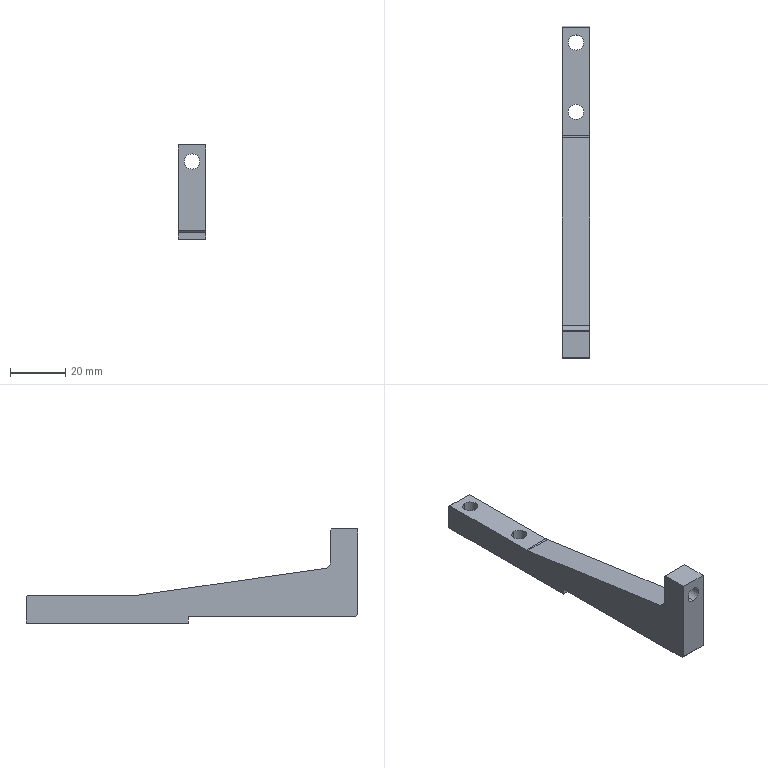Component | SolidWorks | 05-1111-1 | 1 solid | 22 faces | box 10 x 120 x 34 mm | volume 15839 mm3 | plane 14 | cylinder 8 | commonest cylinder face diameters 5.5 x6 4 x1 10 x1
build123d program:
from build123d import *

# Parameters (mm, degrees)
SKETCH1_2_W            = 34
SKETCH1_2_H            = 120
BOSS_EXTRUDE1_DEPTH    = 10
CUT_EXTRUDE1_DEPTH     = 64.159
CHAMFER1_SIZE          = 3
FILLET1_R              = 2
FILLET2_R              = 5
M5_CLEARANCE_HOLE1_D   = 5.5
M5_CLEARANCE_HOLE2_D   = 5.5
CHAMFER2_SIZE          = 0.5
SKETCH1_W              = 2.7
SKETCH1_H              = 62.3
RELIEF_09_FLANGE_DEPTH = 25


with BuildPart() as part:
    # Sketch1_2 → Boss-Extrude1 (new body)
    with BuildSketch(Plane(origin=(0, 0, 0), x_dir=(1, 0, 0), z_dir=(0, 1, 0))):
        Rectangle(SKETCH1_2_W, SKETCH1_2_H)
    extrude(amount=BOSS_EXTRUDE1_DEPTH)

    # Sketch2 → Cut-Extrude1 (cut, through all)
    with BuildSketch(Plane(origin=(0, 10, 0), x_dir=(1, 0, 0), z_dir=(0, 1, 0))):
        Polygon((-7, 60), (-7, 20), (3, -50), (17, -50), (17, 60), align=None)
    extrude(amount=-CUT_EXTRUDE1_DEPTH, mode=Mode.SUBTRACT)

    # Chamfer1
    chamfer1_edges = [part.edges().sort_by_distance(p)[0] for p in [
        (-17, 5, 60),
    ]]
    chamfer(chamfer1_edges, length=CHAMFER1_SIZE)

    # Fillet1
    fillet1_edges = [part.edges().sort_by_distance(p)[0] for p in [
        (3, 5, 50),
    ]]
    fillet(fillet1_edges, radius=FILLET1_R)

    # Fillet2
    fillet2_edges = [part.edges().sort_by_distance(p)[0] for p in [
        (-7, 5, -20),
    ]]
    fillet(fillet2_edges, radius=FILLET2_R)

    # M5 Clearance Hole1 (through all)
    with Locations(Plane.XY.offset(60)):
        with Locations((11, 5)):
            Hole(M5_CLEARANCE_HOLE1_D / 2)

    # M5 Clearance Hole2 (through all)
    with Locations(Plane.ZY.offset(17)):
        with Locations((-29, 5), (-54, 5)):
            Hole(M5_CLEARANCE_HOLE2_D / 2)

    # Chamfer2
    chamfer2_edges = [part.edges().sort_by_distance(p)[0] for p in [
        (-7, 5, -60),
        (17, 5, 50),
    ]]
    chamfer(chamfer2_edges, length=CHAMFER2_SIZE)

    # Sketch1 → Relief-09-flange (cut, symmetric)
    with BuildSketch(Plane(origin=(0, 0, 0), x_dir=(1, 0, 0), z_dir=(0, 1, 0))):
        with Locations((-16.15, -29.85)):
            Rectangle(SKETCH1_W, SKETCH1_H)
    extrude(amount=RELIEF_09_FLANGE_DEPTH, both=True, mode=Mode.SUBTRACT)


solid = part.part

# Placed as in the assembly
solid = solid.moved(Location((-130.072, 468.224, 1533.056), (90, 0, 90)))
STEP:
#1=COLOUR_RGB('',0.7922,0.8196,0.9333);
#2=FILL_AREA_STYLE_COLOUR('',#1);
#3=FILL_AREA_STYLE('',(#2));
#4=SURFACE_STYLE_FILL_AREA(#3);
#5=SURFACE_SIDE_STYLE('',(#4));
#6=SURFACE_STYLE_USAGE(.BOTH.,#5);
#7=PRESENTATION_STYLE_ASSIGNMENT((#6));
#8=CARTESIAN_POINT('',(-5.318,19.684,60.081));
#9=VERTEX_POINT('',#8);
#10=CARTESIAN_POINT('',(-5.318,19.467,60.081));
#11=VERTEX_POINT('',#10);
#12=CARTESIAN_POINT('',(-5.318,19.576,60.081));
#13=DIRECTION('',(-0.,-0.,-1.));
#14=DIRECTION('',(0.,-1.,0.));
#15=AXIS2_PLACEMENT_3D('',#12,#13,#14);
#16=CIRCLE('',#15,0.1083);
#17=EDGE_CURVE('',#9,#11,#16,.T.);
#18=ORIENTED_EDGE('',*,*,#17,.F.);
#19=CARTESIAN_POINT('',(-5.318,19.684,59.687));
#20=VERTEX_POINT('',#19);
#21=CARTESIAN_POINT('',(-5.318,19.684,59.687));
#22=DIRECTION('',(-0.,-0.,-1.));
#23=VECTOR('',#22,39.37);
#24=LINE('',#21,#23);
#25=EDGE_CURVE('',#9,#20,#24,.T.);
#26=ORIENTED_EDGE('',*,*,#25,.T.);
#27=CARTESIAN_POINT('',(-5.318,19.467,59.687));
#28=VERTEX_POINT('',#27);
#29=CARTESIAN_POINT('',(-5.318,19.576,59.687));
#30=DIRECTION('',(-0.,-0.,-1.));
#31=DIRECTION('',(0.,-1.,0.));
#32=AXIS2_PLACEMENT_3D('',#29,#30,#31);
#33=CIRCLE('',#32,0.1083);
#34=EDGE_CURVE('',#20,#28,#33,.T.);
#35=ORIENTED_EDGE('',*,*,#34,.T.);
#36=CARTESIAN_POINT('',(-5.318,19.467,59.687));
#37=DIRECTION('',(-0.,-0.,-1.));
#38=VECTOR('',#37,39.37);
#39=LINE('',#36,#38);
#40=EDGE_CURVE('',#11,#28,#39,.T.);
#41=ORIENTED_EDGE('',*,*,#40,.F.);
#42=EDGE_LOOP('',(#18,#26,#35,#41));
#43=FACE_OUTER_BOUND('',#42,.T.);
#44=CARTESIAN_POINT('',(-5.318,19.576,59.687));
#45=DIRECTION('',(-0.,-0.,-1.));
#46=DIRECTION('',(0.,-1.,0.));
#47=AXIS2_PLACEMENT_3D('',#44,#45,#46);
#48=CYLINDRICAL_SURFACE('',#47,0.1083);
#49=ADVANCED_FACE('',(#43),#48,.F.);
#50=CARTESIAN_POINT('',(-5.318,20.668,60.081));
#51=VERTEX_POINT('',#50);
#52=CARTESIAN_POINT('',(-5.318,20.452,60.081));
#53=VERTEX_POINT('',#52);
#54=CARTESIAN_POINT('',(-5.318,20.56,60.081));
#55=DIRECTION('',(-0.,-0.,-1.));
#56=DIRECTION('',(0.,-1.,0.));
#57=AXIS2_PLACEMENT_3D('',#54,#55,#56);
#58=CIRCLE('',#57,0.1083);
#59=EDGE_CURVE('',#51,#53,#58,.T.);
#60=ORIENTED_EDGE('',*,*,#59,.F.);
#61=CARTESIAN_POINT('',(-5.318,20.668,59.687));
#62=VERTEX_POINT('',#61);
#63=CARTESIAN_POINT('',(-5.318,20.668,59.687));
#64=DIRECTION('',(-0.,-0.,-1.));
#65=VECTOR('',#64,39.37);
#66=LINE('',#63,#65);
#67=EDGE_CURVE('',#51,#62,#66,.T.);
#68=ORIENTED_EDGE('',*,*,#67,.T.);
#69=CARTESIAN_POINT('',(-5.318,20.452,59.687));
#70=VERTEX_POINT('',#69);
#71=CARTESIAN_POINT('',(-5.318,20.56,59.687));
#72=DIRECTION('',(-0.,-0.,-1.));
#73=DIRECTION('',(0.,-1.,0.));
#74=AXIS2_PLACEMENT_3D('',#71,#72,#73);
#75=CIRCLE('',#74,0.1083);
#76=EDGE_CURVE('',#62,#70,#75,.T.);
#77=ORIENTED_EDGE('',*,*,#76,.T.);
#78=CARTESIAN_POINT('',(-5.318,20.452,59.687));
#79=DIRECTION('',(-0.,-0.,-1.));
#80=VECTOR('',#79,39.37);
#81=LINE('',#78,#80);
#82=EDGE_CURVE('',#53,#70,#81,.T.);
#83=ORIENTED_EDGE('',*,*,#82,.F.);
#84=EDGE_LOOP('',(#60,#68,#77,#83));
#85=FACE_OUTER_BOUND('',#84,.T.);
#86=CARTESIAN_POINT('',(-5.318,20.56,59.687));
#87=DIRECTION('',(-0.,-0.,-1.));
#88=DIRECTION('',(0.,-1.,0.));
#89=AXIS2_PLACEMENT_3D('',#86,#87,#88);
#90=CYLINDRICAL_SURFACE('',#89,0.1083);
#91=ADVANCED_FACE('',(#85),#90,.F.);
#92=CARTESIAN_POINT('',(-5.318,16.466,60.681));
#93=VERTEX_POINT('',#92);
#94=CARTESIAN_POINT('',(-5.318,16.466,60.898));
#95=VERTEX_POINT('',#94);
#96=CARTESIAN_POINT('',(-5.318,16.466,60.79));
#97=DIRECTION('',(-0.,-1.,0.));
#98=DIRECTION('',(0.,0.,1.));
#99=AXIS2_PLACEMENT_3D('',#96,#97,#98);
#100=CIRCLE('',#99,0.1083);
#101=EDGE_CURVE('',#93,#95,#100,.T.);
#102=ORIENTED_EDGE('',*,*,#101,.F.);
#103=CARTESIAN_POINT('',(-5.318,16.072,60.681));
#104=VERTEX_POINT('',#103);
#105=CARTESIAN_POINT('',(-5.318,16.072,60.681));
#106=DIRECTION('',(-0.,-1.,0.));
#107=VECTOR('',#106,39.37);
#108=LINE('',#105,#107);
#109=EDGE_CURVE('',#93,#104,#108,.T.);
#110=ORIENTED_EDGE('',*,*,#109,.T.);
#111=CARTESIAN_POINT('',(-5.318,16.072,60.898));
#112=VERTEX_POINT('',#111);
#113=CARTESIAN_POINT('',(-5.318,16.072,60.79));
#114=DIRECTION('',(-0.,-1.,0.));
#115=DIRECTION('',(0.,0.,1.));
#116=AXIS2_PLACEMENT_3D('',#113,#114,#115);
#117=CIRCLE('',#116,0.1083);
#118=EDGE_CURVE('',#104,#112,#117,.T.);
#119=ORIENTED_EDGE('',*,*,#118,.T.);
#120=CARTESIAN_POINT('',(-5.318,16.072,60.898));
#121=DIRECTION('',(-0.,-1.,0.));
#122=VECTOR('',#121,39.37);
#123=LINE('',#120,#122);
#124=EDGE_CURVE('',#95,#112,#123,.T.);
#125=ORIENTED_EDGE('',*,*,#124,.F.);
#126=EDGE_LOOP('',(#102,#110,#119,#125));
#127=FACE_OUTER_BOUND('',#126,.T.);
#128=CARTESIAN_POINT('',(-5.318,16.072,60.79));
#129=DIRECTION('',(-0.,-1.,0.));
#130=DIRECTION('',(0.,0.,1.));
#131=AXIS2_PLACEMENT_3D('',#128,#129,#130);
#132=CYLINDRICAL_SURFACE('',#131,0.1083);
#133=ADVANCED_FACE('',(#127),#132,.F.);
#134=CARTESIAN_POINT('',(-5.121,16.072,61.026));
#135=VERTEX_POINT('',#134);
#136=CARTESIAN_POINT('',(-5.121,16.446,61.026));
#137=VERTEX_POINT('',#136);
#138=CARTESIAN_POINT('',(-5.121,20.796,61.026));
#139=DIRECTION('',(0.,1.,-0.));
#140=VECTOR('',#139,39.37);
#141=LINE('',#138,#140);
#142=EDGE_CURVE('',#135,#137,#141,.T.);
#143=ORIENTED_EDGE('',*,*,#142,.T.);
#144=CARTESIAN_POINT('',(-5.515,16.446,61.026));
#145=VERTEX_POINT('',#144);
#146=CARTESIAN_POINT('',(-5.515,16.446,61.026));
#147=DIRECTION('',(-1.,0.,0.));
#148=VECTOR('',#147,39.37);
#149=LINE('',#146,#148);
#150=EDGE_CURVE('',#137,#145,#149,.T.);
#151=ORIENTED_EDGE('',*,*,#150,.T.);
#152=CARTESIAN_POINT('',(-5.515,16.072,61.026));
#153=VERTEX_POINT('',#152);
#154=CARTESIAN_POINT('',(-5.515,20.796,61.026));
#155=DIRECTION('',(0.,1.,-0.));
#156=VECTOR('',#155,39.37);
#157=LINE('',#154,#156);
#158=EDGE_CURVE('',#153,#145,#157,.T.);
#159=ORIENTED_EDGE('',*,*,#158,.F.);
#160=CARTESIAN_POINT('',(-5.515,16.072,61.026));
#161=DIRECTION('',(1.,-0.,0.));
#162=VECTOR('',#161,39.37);
#163=LINE('',#160,#162);
#164=EDGE_CURVE('',#153,#135,#163,.T.);
#165=ORIENTED_EDGE('',*,*,#164,.T.);
#166=EDGE_LOOP('',(#143,#151,#159,#165));
#167=FACE_OUTER_BOUND('',#166,.T.);
#168=CARTESIAN_POINT('',(-5.515,20.796,61.026));
#169=DIRECTION('',(-0.,-0.,-1.));
#170=DIRECTION('',(-0.,-1.,0.));
#171=AXIS2_PLACEMENT_3D('',#168,#169,#170);
#172=PLANE('',#171);
#173=ADVANCED_FACE('',(#167),#172,.F.);
#174=CARTESIAN_POINT('',(-5.515,20.796,60.061));
#175=VERTEX_POINT('',#174);
#176=CARTESIAN_POINT('',(-5.515,20.796,59.687));
#177=VERTEX_POINT('',#176);
#178=CARTESIAN_POINT('',(-5.515,20.796,59.687));
#179=DIRECTION('',(0.,-0.,-1.));
#180=VECTOR('',#179,39.37);
#181=LINE('',#178,#180);
#182=EDGE_CURVE('',#175,#177,#181,.T.);
#183=ORIENTED_EDGE('',*,*,#182,.F.);
#184=CARTESIAN_POINT('',(-5.121,20.796,60.061));
#185=VERTEX_POINT('',#184);
#186=CARTESIAN_POINT('',(-5.515,20.796,60.061));
#187=DIRECTION('',(1.,-0.,0.));
#188=VECTOR('',#187,39.37);
#189=LINE('',#186,#188);
#190=EDGE_CURVE('',#175,#185,#189,.T.);
#191=ORIENTED_EDGE('',*,*,#190,.T.);
#192=CARTESIAN_POINT('',(-5.121,20.796,59.687));
#193=VERTEX_POINT('',#192);
#194=CARTESIAN_POINT('',(-5.121,20.796,59.687));
#195=DIRECTION('',(0.,-0.,-1.));
#196=VECTOR('',#195,39.37);
#197=LINE('',#194,#196);
#198=EDGE_CURVE('',#185,#193,#197,.T.);
#199=ORIENTED_EDGE('',*,*,#198,.T.);
#200=CARTESIAN_POINT('',(-5.515,20.796,59.687));
#201=DIRECTION('',(1.,-0.,0.));
#202=VECTOR('',#201,39.37);
#203=LINE('',#200,#202);
#204=EDGE_CURVE('',#177,#193,#203,.T.);
#205=ORIENTED_EDGE('',*,*,#204,.F.);
#206=EDGE_LOOP('',(#183,#191,#199,#205));
#207=FACE_OUTER_BOUND('',#206,.T.);
#208=CARTESIAN_POINT('',(-5.515,20.796,59.687));
#209=DIRECTION('',(-0.,-1.,0.));
#210=DIRECTION('',(0.,0.,1.));
#211=AXIS2_PLACEMENT_3D('',#208,#209,#210);
#212=PLANE('',#211);
#213=ADVANCED_FACE('',(#207),#212,.F.);
#214=CARTESIAN_POINT('',(-5.318,19.576,59.687));
#215=DIRECTION('',(-0.,-0.,-1.));
#216=DIRECTION('',(0.,-1.,0.));
#217=AXIS2_PLACEMENT_3D('',#214,#215,#216);
#218=CIRCLE('',#217,0.1083);
#219=EDGE_CURVE('',#28,#20,#218,.T.);
#220=ORIENTED_EDGE('',*,*,#219,.F.);
#221=ORIENTED_EDGE('',*,*,#34,.F.);
#222=EDGE_LOOP('',(#220,#221));
#223=FACE_BOUND('',#222,.T.);
#224=CARTESIAN_POINT('',(-5.318,20.56,59.687));
#225=DIRECTION('',(-0.,-0.,-1.));
#226=DIRECTION('',(0.,-1.,0.));
#227=AXIS2_PLACEMENT_3D('',#224,#225,#226);
#228=CIRCLE('',#227,0.1083);
#229=EDGE_CURVE('',#70,#62,#228,.T.);
#230=ORIENTED_EDGE('',*,*,#229,.F.);
#231=ORIENTED_EDGE('',*,*,#76,.F.);
#232=EDGE_LOOP('',(#230,#231));
#233=FACE_BOUND('',#232,.T.);
#234=CARTESIAN_POINT('',(-5.121,18.485,59.687));
#235=VERTEX_POINT('',#234);
#236=CARTESIAN_POINT('',(-5.121,20.796,59.687));
#237=DIRECTION('',(-0.,-1.,0.));
#238=VECTOR('',#237,39.37);
#239=LINE('',#236,#238);
#240=EDGE_CURVE('',#193,#235,#239,.T.);
#241=ORIENTED_EDGE('',*,*,#240,.T.);
#242=CARTESIAN_POINT('',(-5.515,18.485,59.687));
#243=VERTEX_POINT('',#242);
#244=CARTESIAN_POINT('',(-5.515,18.485,59.687));
#245=DIRECTION('',(-1.,0.,0.));
#246=VECTOR('',#245,39.37);
#247=LINE('',#244,#246);
#248=EDGE_CURVE('',#235,#243,#247,.T.);
#249=ORIENTED_EDGE('',*,*,#248,.T.);
#250=CARTESIAN_POINT('',(-5.515,20.796,59.687));
#251=DIRECTION('',(-0.,-1.,0.));
#252=VECTOR('',#251,39.37);
#253=LINE('',#250,#252);
#254=EDGE_CURVE('',#177,#243,#253,.T.);
#255=ORIENTED_EDGE('',*,*,#254,.F.);
#256=ORIENTED_EDGE('',*,*,#204,.T.);
#257=EDGE_LOOP('',(#241,#249,#255,#256));
#258=FACE_OUTER_BOUND('',#257,.T.);
#259=CARTESIAN_POINT('',(-5.515,20.796,59.687));
#260=DIRECTION('',(0.,0.,1.));
#261=DIRECTION('',(0.,1.,-0.));
#262=AXIS2_PLACEMENT_3D('',#259,#260,#261);
#263=PLANE('',#262);
#264=ADVANCED_FACE('',(#223,#233,#258),#263,.F.);
#265=CARTESIAN_POINT('',(-5.318,16.072,60.79));
#266=DIRECTION('',(-0.,-1.,0.));
#267=DIRECTION('',(0.,0.,1.));
#268=AXIS2_PLACEMENT_3D('',#265,#266,#267);
#269=CIRCLE('',#268,0.1083);
#270=EDGE_CURVE('',#112,#104,#269,.T.);
#271=ORIENTED_EDGE('',*,*,#270,.F.);
#272=ORIENTED_EDGE('',*,*,#118,.F.);
#273=EDGE_LOOP('',(#271,#272));
#274=FACE_BOUND('',#273,.T.);
#275=CARTESIAN_POINT('',(-5.515,16.072,59.805));
#276=VERTEX_POINT('',#275);
#277=CARTESIAN_POINT('',(-5.515,16.072,59.687));
#278=DIRECTION('',(0.,0.,1.));
#279=VECTOR('',#278,39.37);
#280=LINE('',#277,#279);
#281=EDGE_CURVE('',#276,#153,#280,.T.);
#282=ORIENTED_EDGE('',*,*,#281,.F.);
#283=CARTESIAN_POINT('',(-5.121,16.072,59.805));
#284=VERTEX_POINT('',#283);
#285=CARTESIAN_POINT('',(-5.515,16.072,59.805));
#286=DIRECTION('',(1.,-0.,0.));
#287=VECTOR('',#286,39.37);
#288=LINE('',#285,#287);
#289=EDGE_CURVE('',#276,#284,#288,.T.);
#290=ORIENTED_EDGE('',*,*,#289,.T.);
#291=CARTESIAN_POINT('',(-5.121,16.072,59.687));
#292=DIRECTION('',(0.,0.,1.));
#293=VECTOR('',#292,39.37);
#294=LINE('',#291,#293);
#295=EDGE_CURVE('',#284,#135,#294,.T.);
#296=ORIENTED_EDGE('',*,*,#295,.T.);
#297=ORIENTED_EDGE('',*,*,#164,.F.);
#298=EDGE_LOOP('',(#282,#290,#296,#297));
#299=FACE_OUTER_BOUND('',#298,.T.);
#300=CARTESIAN_POINT('',(-5.515,16.072,59.687));
#301=DIRECTION('',(0.,1.,-0.));
#302=DIRECTION('',(0.,-0.,-1.));
#303=AXIS2_PLACEMENT_3D('',#300,#301,#302);
#304=PLANE('',#303);
#305=ADVANCED_FACE('',(#274,#299),#304,.F.);
#306=CARTESIAN_POINT('',(-5.515,18.485,59.774));
#307=VERTEX_POINT('',#306);
#308=CARTESIAN_POINT('',(-5.515,18.485,60.357));
#309=DIRECTION('',(0.,-0.,-1.));
#310=VECTOR('',#309,39.37);
#311=LINE('',#308,#310);
#312=EDGE_CURVE('',#307,#243,#311,.T.);
#313=ORIENTED_EDGE('',*,*,#312,.F.);
#314=CARTESIAN_POINT('',(-5.515,16.103,59.774));
#315=VERTEX_POINT('',#314);
#316=CARTESIAN_POINT('',(-5.515,18.434,59.774));
#317=DIRECTION('',(0.,1.,-0.));
#318=VECTOR('',#317,39.37);
#319=LINE('',#316,#318);
#320=EDGE_CURVE('',#315,#307,#319,.T.);
#321=ORIENTED_EDGE('',*,*,#320,.F.);
#322=CARTESIAN_POINT('',(-5.515,16.977,58.9));
#323=DIRECTION('',(-0.,-0.7071,0.7071));
#324=VECTOR('',#323,39.37);
#325=LINE('',#322,#324);
#326=EDGE_CURVE('',#315,#276,#325,.T.);
#327=ORIENTED_EDGE('',*,*,#326,.T.);
#328=ORIENTED_EDGE('',*,*,#281,.T.);
#329=ORIENTED_EDGE('',*,*,#158,.T.);
#330=CARTESIAN_POINT('',(-5.515,16.466,61.006));
#331=VERTEX_POINT('',#330);
#332=CARTESIAN_POINT('',(-5.515,17.775,59.697));
#333=DIRECTION('',(0.,0.7071,-0.7071));
#334=VECTOR('',#333,39.37);
#335=LINE('',#332,#334);
#336=EDGE_CURVE('',#145,#331,#335,.T.);
#337=ORIENTED_EDGE('',*,*,#336,.T.);
#338=CARTESIAN_POINT('',(-5.515,16.466,60.543));
#339=VERTEX_POINT('',#338);
#340=CARTESIAN_POINT('',(-5.515,16.466,60.475));
#341=DIRECTION('',(0.,0.,1.));
#342=VECTOR('',#341,39.37);
#343=LINE('',#340,#342);
#344=EDGE_CURVE('',#339,#331,#343,.T.);
#345=ORIENTED_EDGE('',*,*,#344,.F.);
#346=CARTESIAN_POINT('',(-5.515,16.533,60.465));
#347=VERTEX_POINT('',#346);
#348=CARTESIAN_POINT('',(-5.515,16.544,60.543));
#349=DIRECTION('',(1.,-0.,0.));
#350=DIRECTION('',(0.,-1.,0.));
#351=AXIS2_PLACEMENT_3D('',#348,#349,#350);
#352=CIRCLE('',#351,0.07874);
#353=EDGE_CURVE('',#339,#347,#352,.T.);
#354=ORIENTED_EDGE('',*,*,#353,.T.);
#355=CARTESIAN_POINT('',(-5.515,19.208,60.083));
#356=VERTEX_POINT('',#355);
#357=CARTESIAN_POINT('',(-5.515,19.221,60.081));
#358=DIRECTION('',(-0.,-0.9899,0.1414));
#359=VECTOR('',#358,39.37);
#360=LINE('',#357,#359);
#361=EDGE_CURVE('',#356,#347,#360,.T.);
#362=ORIENTED_EDGE('',*,*,#361,.F.);
#363=CARTESIAN_POINT('',(-5.515,19.235,60.081));
#364=VERTEX_POINT('',#363);
#365=CARTESIAN_POINT('',(-5.515,19.235,60.278));
#366=DIRECTION('',(1.,-0.,0.));
#367=DIRECTION('',(0.,-1.,0.));
#368=AXIS2_PLACEMENT_3D('',#365,#366,#367);
#369=CIRCLE('',#368,0.1969);
#370=EDGE_CURVE('',#356,#364,#369,.T.);
#371=ORIENTED_EDGE('',*,*,#370,.T.);
#372=CARTESIAN_POINT('',(-5.515,20.777,60.081));
#373=VERTEX_POINT('',#372);
#374=CARTESIAN_POINT('',(-5.515,20.796,60.081));
#375=DIRECTION('',(-0.,-1.,0.));
#376=VECTOR('',#375,39.37);
#377=LINE('',#374,#376);
#378=EDGE_CURVE('',#373,#364,#377,.T.);
#379=ORIENTED_EDGE('',*,*,#378,.F.);
#380=CARTESIAN_POINT('',(-5.515,19.467,61.39));
#381=DIRECTION('',(0.,0.7071,-0.7071));
#382=VECTOR('',#381,39.37);
#383=LINE('',#380,#382);
#384=EDGE_CURVE('',#373,#175,#383,.T.);
#385=ORIENTED_EDGE('',*,*,#384,.T.);
#386=ORIENTED_EDGE('',*,*,#182,.T.);
#387=ORIENTED_EDGE('',*,*,#254,.T.);
#388=EDGE_LOOP('',(#313,#321,#327,#328,#329,#337,#345,#354,#362,#371,#379,#385,#386,#387));
#389=FACE_OUTER_BOUND('',#388,.T.);
#390=CARTESIAN_POINT('',(-5.515,18.434,60.357));
#391=DIRECTION('',(-1.,0.,0.));
#392=DIRECTION('',(-0.,-1.,0.));
#393=AXIS2_PLACEMENT_3D('',#390,#391,#392);
#394=PLANE('',#393);
#395=ADVANCED_FACE('',(#389),#394,.T.);
#396=CARTESIAN_POINT('',(-5.121,16.103,59.774));
#397=VERTEX_POINT('',#396);
#398=CARTESIAN_POINT('',(-5.121,18.485,59.774));
#399=VERTEX_POINT('',#398);
#400=CARTESIAN_POINT('',(-5.121,18.434,59.774));
#401=DIRECTION('',(0.,1.,-0.));
#402=VECTOR('',#401,39.37);
#403=LINE('',#400,#402);
#404=EDGE_CURVE('',#397,#399,#403,.T.);
#405=ORIENTED_EDGE('',*,*,#404,.T.);
#406=CARTESIAN_POINT('',(-5.121,18.485,60.357));
#407=DIRECTION('',(0.,-0.,-1.));
#408=VECTOR('',#407,39.37);
#409=LINE('',#406,#408);
#410=EDGE_CURVE('',#399,#235,#409,.T.);
#411=ORIENTED_EDGE('',*,*,#410,.T.);
#412=ORIENTED_EDGE('',*,*,#240,.F.);
#413=ORIENTED_EDGE('',*,*,#198,.F.);
#414=CARTESIAN_POINT('',(-5.121,20.777,60.081));
#415=VERTEX_POINT('',#414);
#416=CARTESIAN_POINT('',(-5.121,20.777,60.081));
#417=DIRECTION('',(-0.,-0.7071,0.7071));
#418=VECTOR('',#417,39.37);
#419=LINE('',#416,#418);
#420=EDGE_CURVE('',#185,#415,#419,.T.);
#421=ORIENTED_EDGE('',*,*,#420,.T.);
#422=CARTESIAN_POINT('',(-5.121,19.235,60.081));
#423=VERTEX_POINT('',#422);
#424=CARTESIAN_POINT('',(-5.121,20.796,60.081));
#425=DIRECTION('',(-0.,-1.,0.));
#426=VECTOR('',#425,39.37);
#427=LINE('',#424,#426);
#428=EDGE_CURVE('',#415,#423,#427,.T.);
#429=ORIENTED_EDGE('',*,*,#428,.T.);
#430=CARTESIAN_POINT('',(-5.121,19.208,60.083));
#431=VERTEX_POINT('',#430);
#432=CARTESIAN_POINT('',(-5.121,19.235,60.278));
#433=DIRECTION('',(-1.,0.,0.));
#434=DIRECTION('',(0.,-1.,0.));
#435=AXIS2_PLACEMENT_3D('',#432,#433,#434);
#436=CIRCLE('',#435,0.1969);
#437=EDGE_CURVE('',#423,#431,#436,.T.);
#438=ORIENTED_EDGE('',*,*,#437,.T.);
#439=CARTESIAN_POINT('',(-5.121,16.533,60.465));
#440=VERTEX_POINT('',#439);
#441=CARTESIAN_POINT('',(-5.121,19.221,60.081));
#442=DIRECTION('',(-0.,-0.9899,0.1414));
#443=VECTOR('',#442,39.37);
#444=LINE('',#441,#443);
#445=EDGE_CURVE('',#431,#440,#444,.T.);
#446=ORIENTED_EDGE('',*,*,#445,.T.);
#447=CARTESIAN_POINT('',(-5.121,16.466,60.543));
#448=VERTEX_POINT('',#447);
#449=CARTESIAN_POINT('',(-5.121,16.544,60.543));
#450=DIRECTION('',(-1.,0.,0.));
#451=DIRECTION('',(0.,-1.,0.));
#452=AXIS2_PLACEMENT_3D('',#449,#450,#451);
#453=CIRCLE('',#452,0.07874);
#454=EDGE_CURVE('',#440,#448,#453,.T.);
#455=ORIENTED_EDGE('',*,*,#454,.T.);
#456=CARTESIAN_POINT('',(-5.121,16.466,61.006));
#457=VERTEX_POINT('',#456);
#458=CARTESIAN_POINT('',(-5.121,16.466,60.475));
#459=DIRECTION('',(0.,0.,1.));
#460=VECTOR('',#459,39.37);
#461=LINE('',#458,#460);
#462=EDGE_CURVE('',#448,#457,#461,.T.);
#463=ORIENTED_EDGE('',*,*,#462,.T.);
#464=CARTESIAN_POINT('',(-5.121,16.446,61.026));
#465=DIRECTION('',(-0.,-0.7071,0.7071));
#466=VECTOR('',#465,39.37);
#467=LINE('',#464,#466);
#468=EDGE_CURVE('',#457,#137,#467,.T.);
#469=ORIENTED_EDGE('',*,*,#468,.T.);
#470=ORIENTED_EDGE('',*,*,#142,.F.);
#471=ORIENTED_EDGE('',*,*,#295,.F.);
#472=CARTESIAN_POINT('',(-5.121,16.072,59.805));
#473=DIRECTION('',(0.,0.7071,-0.7071));
#474=VECTOR('',#473,39.37);
#475=LINE('',#472,#474);
#476=EDGE_CURVE('',#284,#397,#475,.T.);
#477=ORIENTED_EDGE('',*,*,#476,.T.);
#478=EDGE_LOOP('',(#405,#411,#412,#413,#421,#429,#438,#446,#455,#463,#469,#470,#471,#477));
#479=FACE_OUTER_BOUND('',#478,.T.);
#480=CARTESIAN_POINT('',(-5.121,18.434,60.357));
#481=DIRECTION('',(-1.,0.,0.));
#482=DIRECTION('',(-0.,-1.,0.));
#483=AXIS2_PLACEMENT_3D('',#480,#481,#482);
#484=PLANE('',#483);
#485=ADVANCED_FACE('',(#479),#484,.F.);
#486=CARTESIAN_POINT('',(-5.318,16.466,60.79));
#487=DIRECTION('',(-0.,-1.,0.));
#488=DIRECTION('',(0.,0.,1.));
#489=AXIS2_PLACEMENT_3D('',#486,#487,#488);
#490=CIRCLE('',#489,0.1083);
#491=EDGE_CURVE('',#95,#93,#490,.T.);
#492=ORIENTED_EDGE('',*,*,#491,.T.);
#493=ORIENTED_EDGE('',*,*,#101,.T.);
#494=EDGE_LOOP('',(#492,#493));
#495=FACE_BOUND('',#494,.T.);
#496=ORIENTED_EDGE('',*,*,#344,.T.);
#497=CARTESIAN_POINT('',(-5.121,16.466,61.006));
#498=DIRECTION('',(1.,-0.,0.));
#499=VECTOR('',#498,39.37);
#500=LINE('',#497,#499);
#501=EDGE_CURVE('',#331,#457,#500,.T.);
#502=ORIENTED_EDGE('',*,*,#501,.T.);
#503=ORIENTED_EDGE('',*,*,#462,.F.);
#504=CARTESIAN_POINT('',(-5.515,16.466,60.543));
#505=DIRECTION('',(-1.,0.,0.));
#506=VECTOR('',#505,39.37);
#507=LINE('',#504,#506);
#508=EDGE_CURVE('',#448,#339,#507,.T.);
#509=ORIENTED_EDGE('',*,*,#508,.T.);
#510=EDGE_LOOP('',(#496,#502,#503,#509));
#511=FACE_OUTER_BOUND('',#510,.T.);
#512=CARTESIAN_POINT('',(-5.121,16.466,60.475));
#513=DIRECTION('',(-0.,-1.,0.));
#514=DIRECTION('',(0.,0.,1.));
#515=AXIS2_PLACEMENT_3D('',#512,#513,#514);
#516=PLANE('',#515);
#517=ADVANCED_FACE('',(#495,#511),#516,.F.);
#518=ORIENTED_EDGE('',*,*,#445,.F.);
#519=CARTESIAN_POINT('',(-5.515,19.208,60.083));
#520=DIRECTION('',(-1.,0.,0.));
#521=VECTOR('',#520,39.37);
#522=LINE('',#519,#521);
#523=EDGE_CURVE('',#431,#356,#522,.T.);
#524=ORIENTED_EDGE('',*,*,#523,.T.);
#525=ORIENTED_EDGE('',*,*,#361,.T.);
#526=CARTESIAN_POINT('',(-5.121,16.533,60.465));
#527=DIRECTION('',(1.,-0.,0.));
#528=VECTOR('',#527,39.37);
#529=LINE('',#526,#528);
#530=EDGE_CURVE('',#347,#440,#529,.T.);
#531=ORIENTED_EDGE('',*,*,#530,.T.);
#532=EDGE_LOOP('',(#518,#524,#525,#531));
#533=FACE_OUTER_BOUND('',#532,.T.);
#534=CARTESIAN_POINT('',(-5.121,19.221,60.081));
#535=DIRECTION('',(-0.,-0.1414,-0.9899));
#536=DIRECTION('',(-0.,-0.9899,0.1414));
#537=AXIS2_PLACEMENT_3D('',#534,#535,#536);
#538=PLANE('',#537);
#539=ADVANCED_FACE('',(#533),#538,.F.);
#540=CARTESIAN_POINT('',(-5.318,19.576,60.081));
#541=DIRECTION('',(-0.,-0.,-1.));
#542=DIRECTION('',(0.,-1.,0.));
#543=AXIS2_PLACEMENT_3D('',#540,#541,#542);
#544=CIRCLE('',#543,0.1083);
#545=EDGE_CURVE('',#11,#9,#544,.T.);
#546=ORIENTED_EDGE('',*,*,#545,.T.);
#547=ORIENTED_EDGE('',*,*,#17,.T.);
#548=EDGE_LOOP('',(#546,#547));
#549=FACE_BOUND('',#548,.T.);
#550=CARTESIAN_POINT('',(-5.318,20.56,60.081));
#551=DIRECTION('',(-0.,-0.,-1.));
#552=DIRECTION('',(0.,-1.,0.));
#553=AXIS2_PLACEMENT_3D('',#550,#551,#552);
#554=CIRCLE('',#553,0.1083);
#555=EDGE_CURVE('',#53,#51,#554,.T.);
#556=ORIENTED_EDGE('',*,*,#555,.T.);
#557=ORIENTED_EDGE('',*,*,#59,.T.);
#558=EDGE_LOOP('',(#556,#557));
#559=FACE_BOUND('',#558,.T.);
#560=ORIENTED_EDGE('',*,*,#428,.F.);
#561=CARTESIAN_POINT('',(-5.121,20.777,60.081));
#562=DIRECTION('',(-1.,0.,0.));
#563=VECTOR('',#562,39.37);
#564=LINE('',#561,#563);
#565=EDGE_CURVE('',#415,#373,#564,.T.);
#566=ORIENTED_EDGE('',*,*,#565,.T.);
#567=ORIENTED_EDGE('',*,*,#378,.T.);
#568=CARTESIAN_POINT('',(-5.121,19.235,60.081));
#569=DIRECTION('',(1.,-0.,0.));
#570=VECTOR('',#569,39.37);
#571=LINE('',#568,#570);
#572=EDGE_CURVE('',#364,#423,#571,.T.);
#573=ORIENTED_EDGE('',*,*,#572,.T.);
#574=EDGE_LOOP('',(#560,#566,#567,#573));
#575=FACE_OUTER_BOUND('',#574,.T.);
#576=CARTESIAN_POINT('',(-5.121,20.796,60.081));
#577=DIRECTION('',(-0.,-0.,-1.));
#578=DIRECTION('',(-0.,-1.,0.));
#579=AXIS2_PLACEMENT_3D('',#576,#577,#578);
#580=PLANE('',#579);
#581=ADVANCED_FACE('',(#549,#559,#575),#580,.F.);
#582=CARTESIAN_POINT('',(-5.515,16.103,59.774));
#583=DIRECTION('',(-1.,0.,0.));
#584=VECTOR('',#583,39.37);
#585=LINE('',#582,#584);
#586=EDGE_CURVE('',#397,#315,#585,.T.);
#587=ORIENTED_EDGE('',*,*,#586,.F.);
#588=ORIENTED_EDGE('',*,*,#476,.F.);
#589=ORIENTED_EDGE('',*,*,#289,.F.);
#590=ORIENTED_EDGE('',*,*,#326,.F.);
#591=EDGE_LOOP('',(#587,#588,#589,#590));
#592=FACE_OUTER_BOUND('',#591,.T.);
#593=CARTESIAN_POINT('',(-5.515,16.072,59.805));
#594=DIRECTION('',(0.,0.7071,0.7071));
#595=DIRECTION('',(1.,-0.,0.));
#596=AXIS2_PLACEMENT_3D('',#593,#594,#595);
#597=PLANE('',#596);
#598=ADVANCED_FACE('',(#592),#597,.F.);
#599=ORIENTED_EDGE('',*,*,#454,.F.);
#600=ORIENTED_EDGE('',*,*,#530,.F.);
#601=ORIENTED_EDGE('',*,*,#353,.F.);
#602=ORIENTED_EDGE('',*,*,#508,.F.);
#603=EDGE_LOOP('',(#599,#600,#601,#602));
#604=FACE_OUTER_BOUND('',#603,.T.);
#605=CARTESIAN_POINT('',(-5.121,16.544,60.543));
#606=DIRECTION('',(1.,-0.,0.));
#607=DIRECTION('',(0.,1.,0.));
#608=AXIS2_PLACEMENT_3D('',#605,#606,#607);
#609=CYLINDRICAL_SURFACE('',#608,0.07874);
#610=ADVANCED_FACE('',(#604),#609,.F.);
#611=ORIENTED_EDGE('',*,*,#437,.F.);
#612=ORIENTED_EDGE('',*,*,#572,.F.);
#613=ORIENTED_EDGE('',*,*,#370,.F.);
#614=ORIENTED_EDGE('',*,*,#523,.F.);
#615=EDGE_LOOP('',(#611,#612,#613,#614));
#616=FACE_OUTER_BOUND('',#615,.T.);
#617=CARTESIAN_POINT('',(-5.121,19.235,60.278));
#618=DIRECTION('',(1.,-0.,0.));
#619=DIRECTION('',(0.,1.,0.));
#620=AXIS2_PLACEMENT_3D('',#617,#618,#619);
#621=CYLINDRICAL_SURFACE('',#620,0.1969);
#622=ADVANCED_FACE('',(#616),#621,.F.);
#623=ORIENTED_EDGE('',*,*,#109,.F.);
#624=ORIENTED_EDGE('',*,*,#491,.F.);
#625=ORIENTED_EDGE('',*,*,#124,.T.);
#626=ORIENTED_EDGE('',*,*,#270,.T.);
#627=EDGE_LOOP('',(#623,#624,#625,#626));
#628=FACE_OUTER_BOUND('',#627,.T.);
#629=CARTESIAN_POINT('',(-5.318,16.072,60.79));
#630=DIRECTION('',(-0.,-1.,0.));
#631=DIRECTION('',(0.,0.,1.));
#632=AXIS2_PLACEMENT_3D('',#629,#630,#631);
#633=CYLINDRICAL_SURFACE('',#632,0.1083);
#634=ADVANCED_FACE('',(#628),#633,.F.);
#635=ORIENTED_EDGE('',*,*,#67,.F.);
#636=ORIENTED_EDGE('',*,*,#555,.F.);
#637=ORIENTED_EDGE('',*,*,#82,.T.);
#638=ORIENTED_EDGE('',*,*,#229,.T.);
#639=EDGE_LOOP('',(#635,#636,#637,#638));
#640=FACE_OUTER_BOUND('',#639,.T.);
#641=CARTESIAN_POINT('',(-5.318,20.56,59.687));
#642=DIRECTION('',(-0.,-0.,-1.));
#643=DIRECTION('',(0.,-1.,0.));
#644=AXIS2_PLACEMENT_3D('',#641,#642,#643);
#645=CYLINDRICAL_SURFACE('',#644,0.1083);
#646=ADVANCED_FACE('',(#640),#645,.F.);
#647=ORIENTED_EDGE('',*,*,#25,.F.);
#648=ORIENTED_EDGE('',*,*,#545,.F.);
#649=ORIENTED_EDGE('',*,*,#40,.T.);
#650=ORIENTED_EDGE('',*,*,#219,.T.);
#651=EDGE_LOOP('',(#647,#648,#649,#650));
#652=FACE_OUTER_BOUND('',#651,.T.);
#653=CARTESIAN_POINT('',(-5.318,19.576,59.687));
#654=DIRECTION('',(-0.,-0.,-1.));
#655=DIRECTION('',(0.,-1.,0.));
#656=AXIS2_PLACEMENT_3D('',#653,#654,#655);
#657=CYLINDRICAL_SURFACE('',#656,0.1083);
#658=ADVANCED_FACE('',(#652),#657,.F.);
#659=ORIENTED_EDGE('',*,*,#468,.F.);
#660=ORIENTED_EDGE('',*,*,#501,.F.);
#661=ORIENTED_EDGE('',*,*,#336,.F.);
#662=ORIENTED_EDGE('',*,*,#150,.F.);
#663=EDGE_LOOP('',(#659,#660,#661,#662));
#664=FACE_OUTER_BOUND('',#663,.T.);
#665=CARTESIAN_POINT('',(-5.515,16.446,61.026));
#666=DIRECTION('',(-0.,-0.7071,-0.7071));
#667=DIRECTION('',(-1.,0.,0.));
#668=AXIS2_PLACEMENT_3D('',#665,#666,#667);
#669=PLANE('',#668);
#670=ADVANCED_FACE('',(#664),#669,.F.);
#671=ORIENTED_EDGE('',*,*,#420,.F.);
#672=ORIENTED_EDGE('',*,*,#190,.F.);
#673=ORIENTED_EDGE('',*,*,#384,.F.);
#674=ORIENTED_EDGE('',*,*,#565,.F.);
#675=EDGE_LOOP('',(#671,#672,#673,#674));
#676=FACE_OUTER_BOUND('',#675,.T.);
#677=CARTESIAN_POINT('',(-5.121,20.777,60.081));
#678=DIRECTION('',(-0.,-0.7071,-0.7071));
#679=DIRECTION('',(-1.,0.,0.));
#680=AXIS2_PLACEMENT_3D('',#677,#678,#679);
#681=PLANE('',#680);
#682=ADVANCED_FACE('',(#676),#681,.F.);
#683=ORIENTED_EDGE('',*,*,#312,.T.);
#684=ORIENTED_EDGE('',*,*,#248,.F.);
#685=ORIENTED_EDGE('',*,*,#410,.F.);
#686=CARTESIAN_POINT('',(-4.137,18.485,59.774));
#687=DIRECTION('',(-1.,0.,0.));
#688=VECTOR('',#687,39.37);
#689=LINE('',#686,#688);
#690=EDGE_CURVE('',#399,#307,#689,.T.);
#691=ORIENTED_EDGE('',*,*,#690,.T.);
#692=EDGE_LOOP('',(#683,#684,#685,#691));
#693=FACE_OUTER_BOUND('',#692,.T.);
#694=CARTESIAN_POINT('',(-4.137,18.485,59.668));
#695=DIRECTION('',(0.,1.,-0.));
#696=DIRECTION('',(0.,-0.,-1.));
#697=AXIS2_PLACEMENT_3D('',#694,#695,#696);
#698=PLANE('',#697);
#699=ADVANCED_FACE('',(#693),#698,.F.);
#700=ORIENTED_EDGE('',*,*,#320,.T.);
#701=ORIENTED_EDGE('',*,*,#690,.F.);
#702=ORIENTED_EDGE('',*,*,#404,.F.);
#703=ORIENTED_EDGE('',*,*,#586,.T.);
#704=EDGE_LOOP('',(#700,#701,#702,#703));
#705=FACE_OUTER_BOUND('',#704,.T.);
#706=CARTESIAN_POINT('',(-4.137,18.485,59.774));
#707=DIRECTION('',(0.,0.,1.));
#708=DIRECTION('',(0.,1.,-0.));
#709=AXIS2_PLACEMENT_3D('',#706,#707,#708);
#710=PLANE('',#709);
#711=ADVANCED_FACE('',(#705),#710,.F.);
#712=CLOSED_SHELL('',(#49,#91,#133,#173,#213,#264,#305,#395,#485,#517,#539,#581,#598,#610,#622,#634,#646,#658,#670,#682,#699,#711));
#713=MANIFOLD_SOLID_BREP('',#712);
#714=STYLED_ITEM('',(#7),#713);
#715=(LENGTH_UNIT()NAMED_UNIT(*)SI_UNIT($,.METRE.));
#716=LENGTH_MEASURE_WITH_UNIT(LENGTH_MEASURE(0.0254),#715);
#717=DIMENSIONAL_EXPONENTS(1.,0.,0.,0.,0.,0.,0.);
#718=(CONVERSION_BASED_UNIT('',#716)LENGTH_UNIT()NAMED_UNIT(#717));
#719=UNCERTAINTY_MEASURE_WITH_UNIT(LENGTH_MEASURE(0.00001),#718,'','');
#720=(NAMED_UNIT(*)PLANE_ANGLE_UNIT()SI_UNIT($,.RADIAN.));
#721=(NAMED_UNIT(*)SI_UNIT($,.STERADIAN.)SOLID_ANGLE_UNIT());
#722=(GEOMETRIC_REPRESENTATION_CONTEXT(3)GLOBAL_UNCERTAINTY_ASSIGNED_CONTEXT((#719))GLOBAL_UNIT_ASSIGNED_CONTEXT((#718,#720,#721))REPRESENTATION_CONTEXT('',''));
#723=MECHANICAL_DESIGN_GEOMETRIC_PRESENTATION_REPRESENTATION('',(#714),#722);
#724=CARTESIAN_POINT('',(0.,0.,0.));
#725=DIRECTION('',(0.,0.,1.));
#726=DIRECTION('',(1.,0.,0.));
#727=AXIS2_PLACEMENT_3D('',#724,#725,#726);
#728=(LENGTH_UNIT()NAMED_UNIT(*)SI_UNIT($,.METRE.));
#729=LENGTH_MEASURE_WITH_UNIT(LENGTH_MEASURE(0.0254),#728);
#730=DIMENSIONAL_EXPONENTS(1.,0.,0.,0.,0.,0.,0.);
#731=(CONVERSION_BASED_UNIT('',#729)LENGTH_UNIT()NAMED_UNIT(#730));
#732=UNCERTAINTY_MEASURE_WITH_UNIT(LENGTH_MEASURE(0.00001),#731,'','');
#733=(NAMED_UNIT(*)PLANE_ANGLE_UNIT()SI_UNIT($,.RADIAN.));
#734=(NAMED_UNIT(*)SI_UNIT($,.STERADIAN.)SOLID_ANGLE_UNIT());
#735=(GEOMETRIC_REPRESENTATION_CONTEXT(3)GLOBAL_UNCERTAINTY_ASSIGNED_CONTEXT((#732))GLOBAL_UNIT_ASSIGNED_CONTEXT((#731,#733,#734))REPRESENTATION_CONTEXT('',''));
#736=ADVANCED_BREP_SHAPE_REPRESENTATION('',(#713,#727),#735);
#737=PRESENTATION_LAYER_ASSIGNMENT('','',(#714));